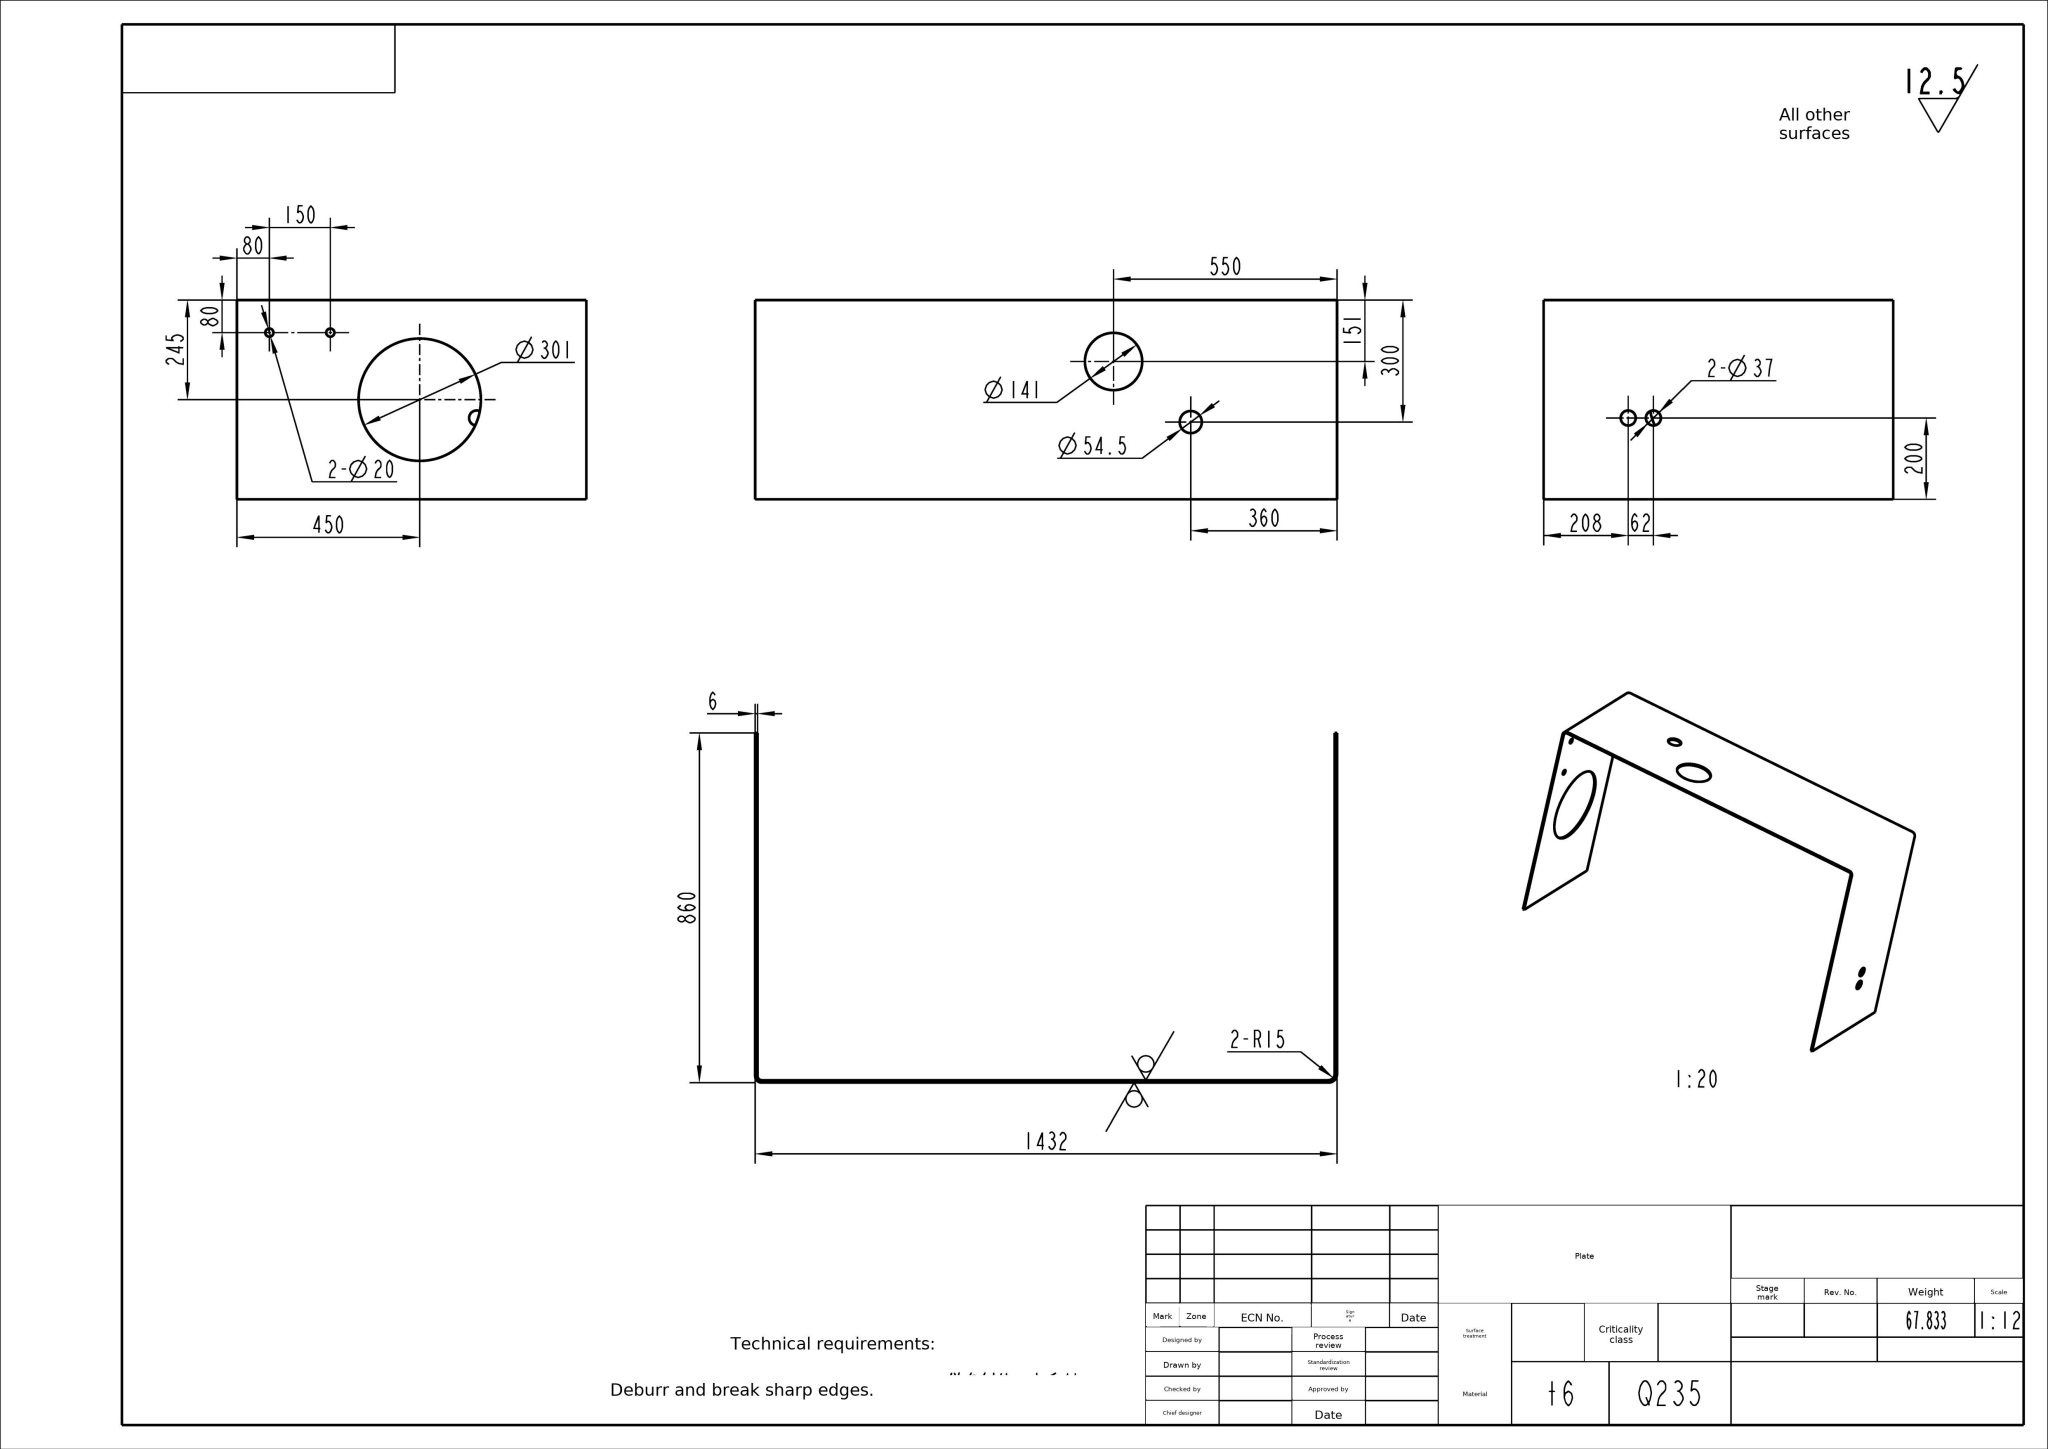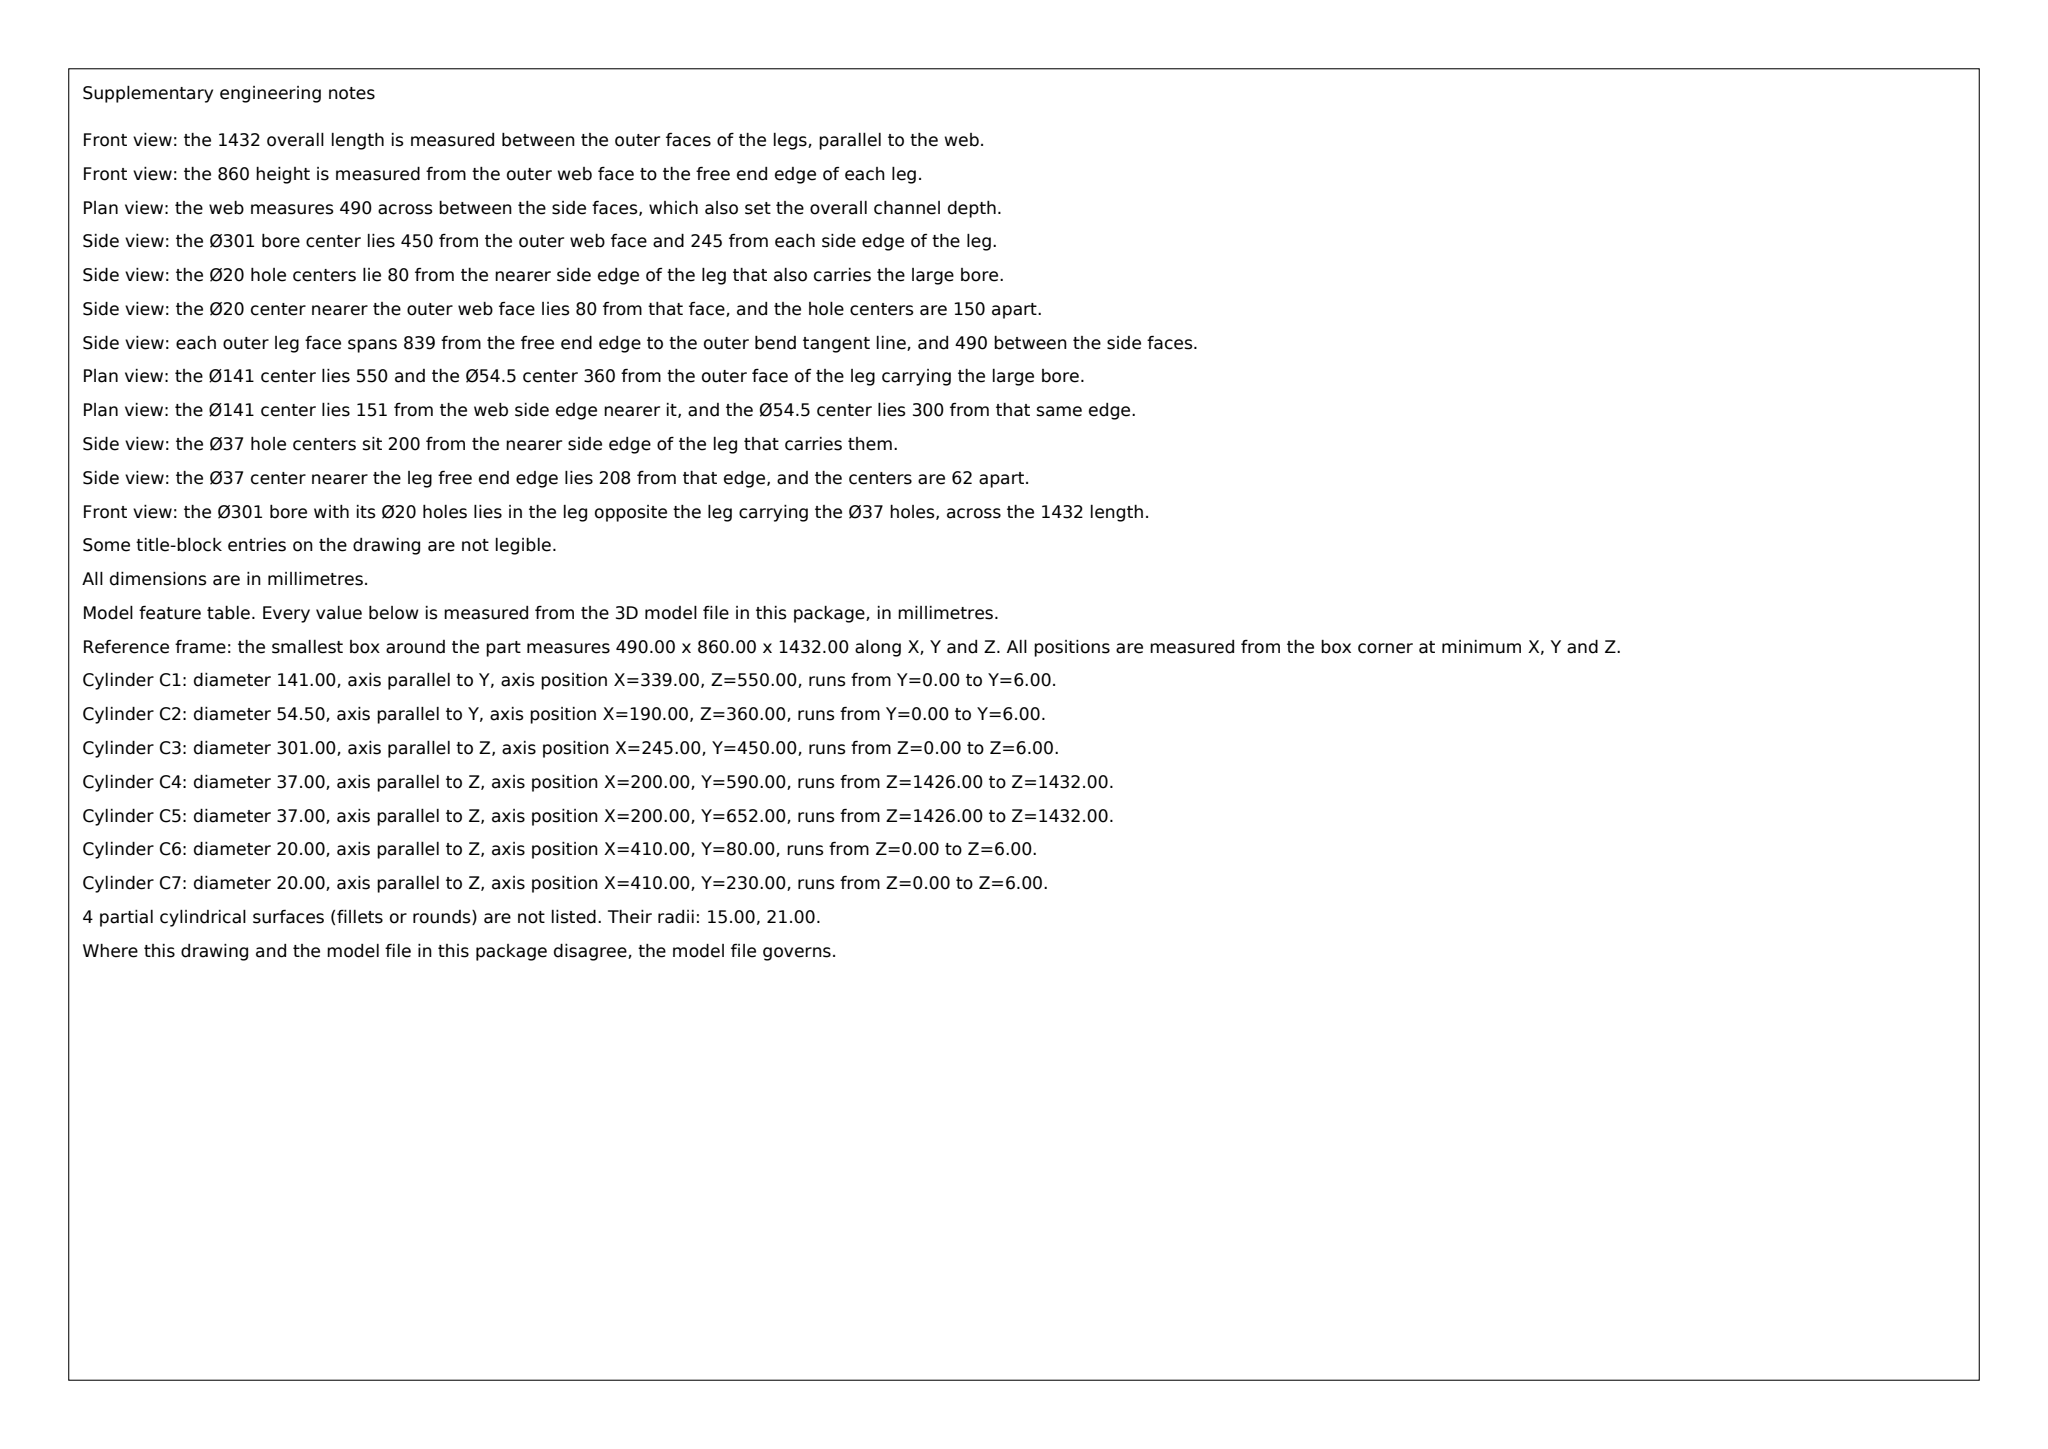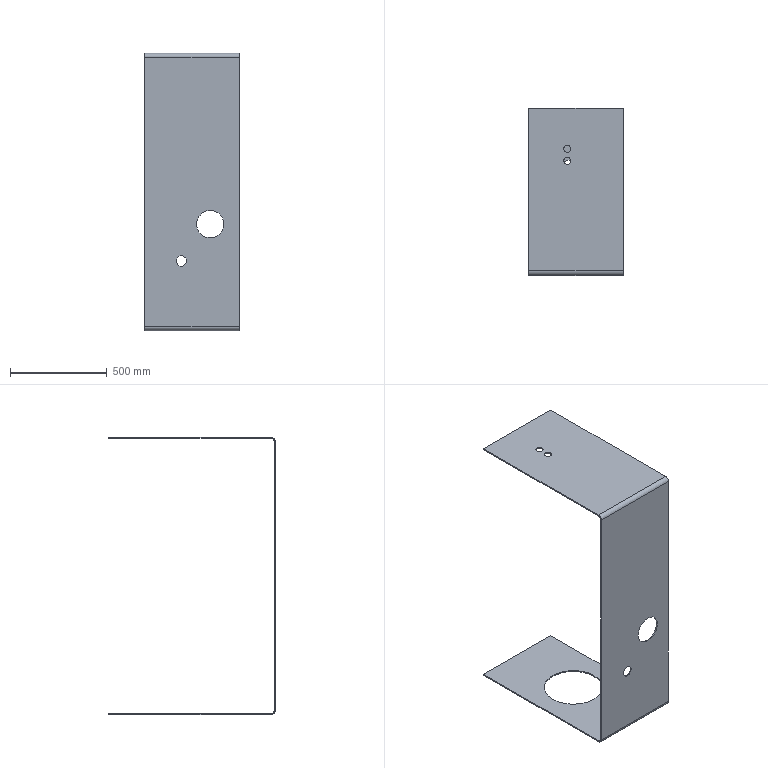Part | SolidWorks | mm | material Q235 | 1 solid | 36 faces | box 490 x 860 x 1432 mm | volume 8634870 mm3 | cylinder 18 | plane 18 | commonest cylinder face diameters 37 x4 20 x4 301 x2 141 x2 54.5 x2 30 x2 42 x2
Drawing notes:
OVERALL WIDTH 490, TYP ALL PANELS (REPLACES 11-490 NOTE) | from the solid: bbox_xyz X = 490.0; planes x=0.0 and x=490.0 bound part; holes dim'd within 490 width